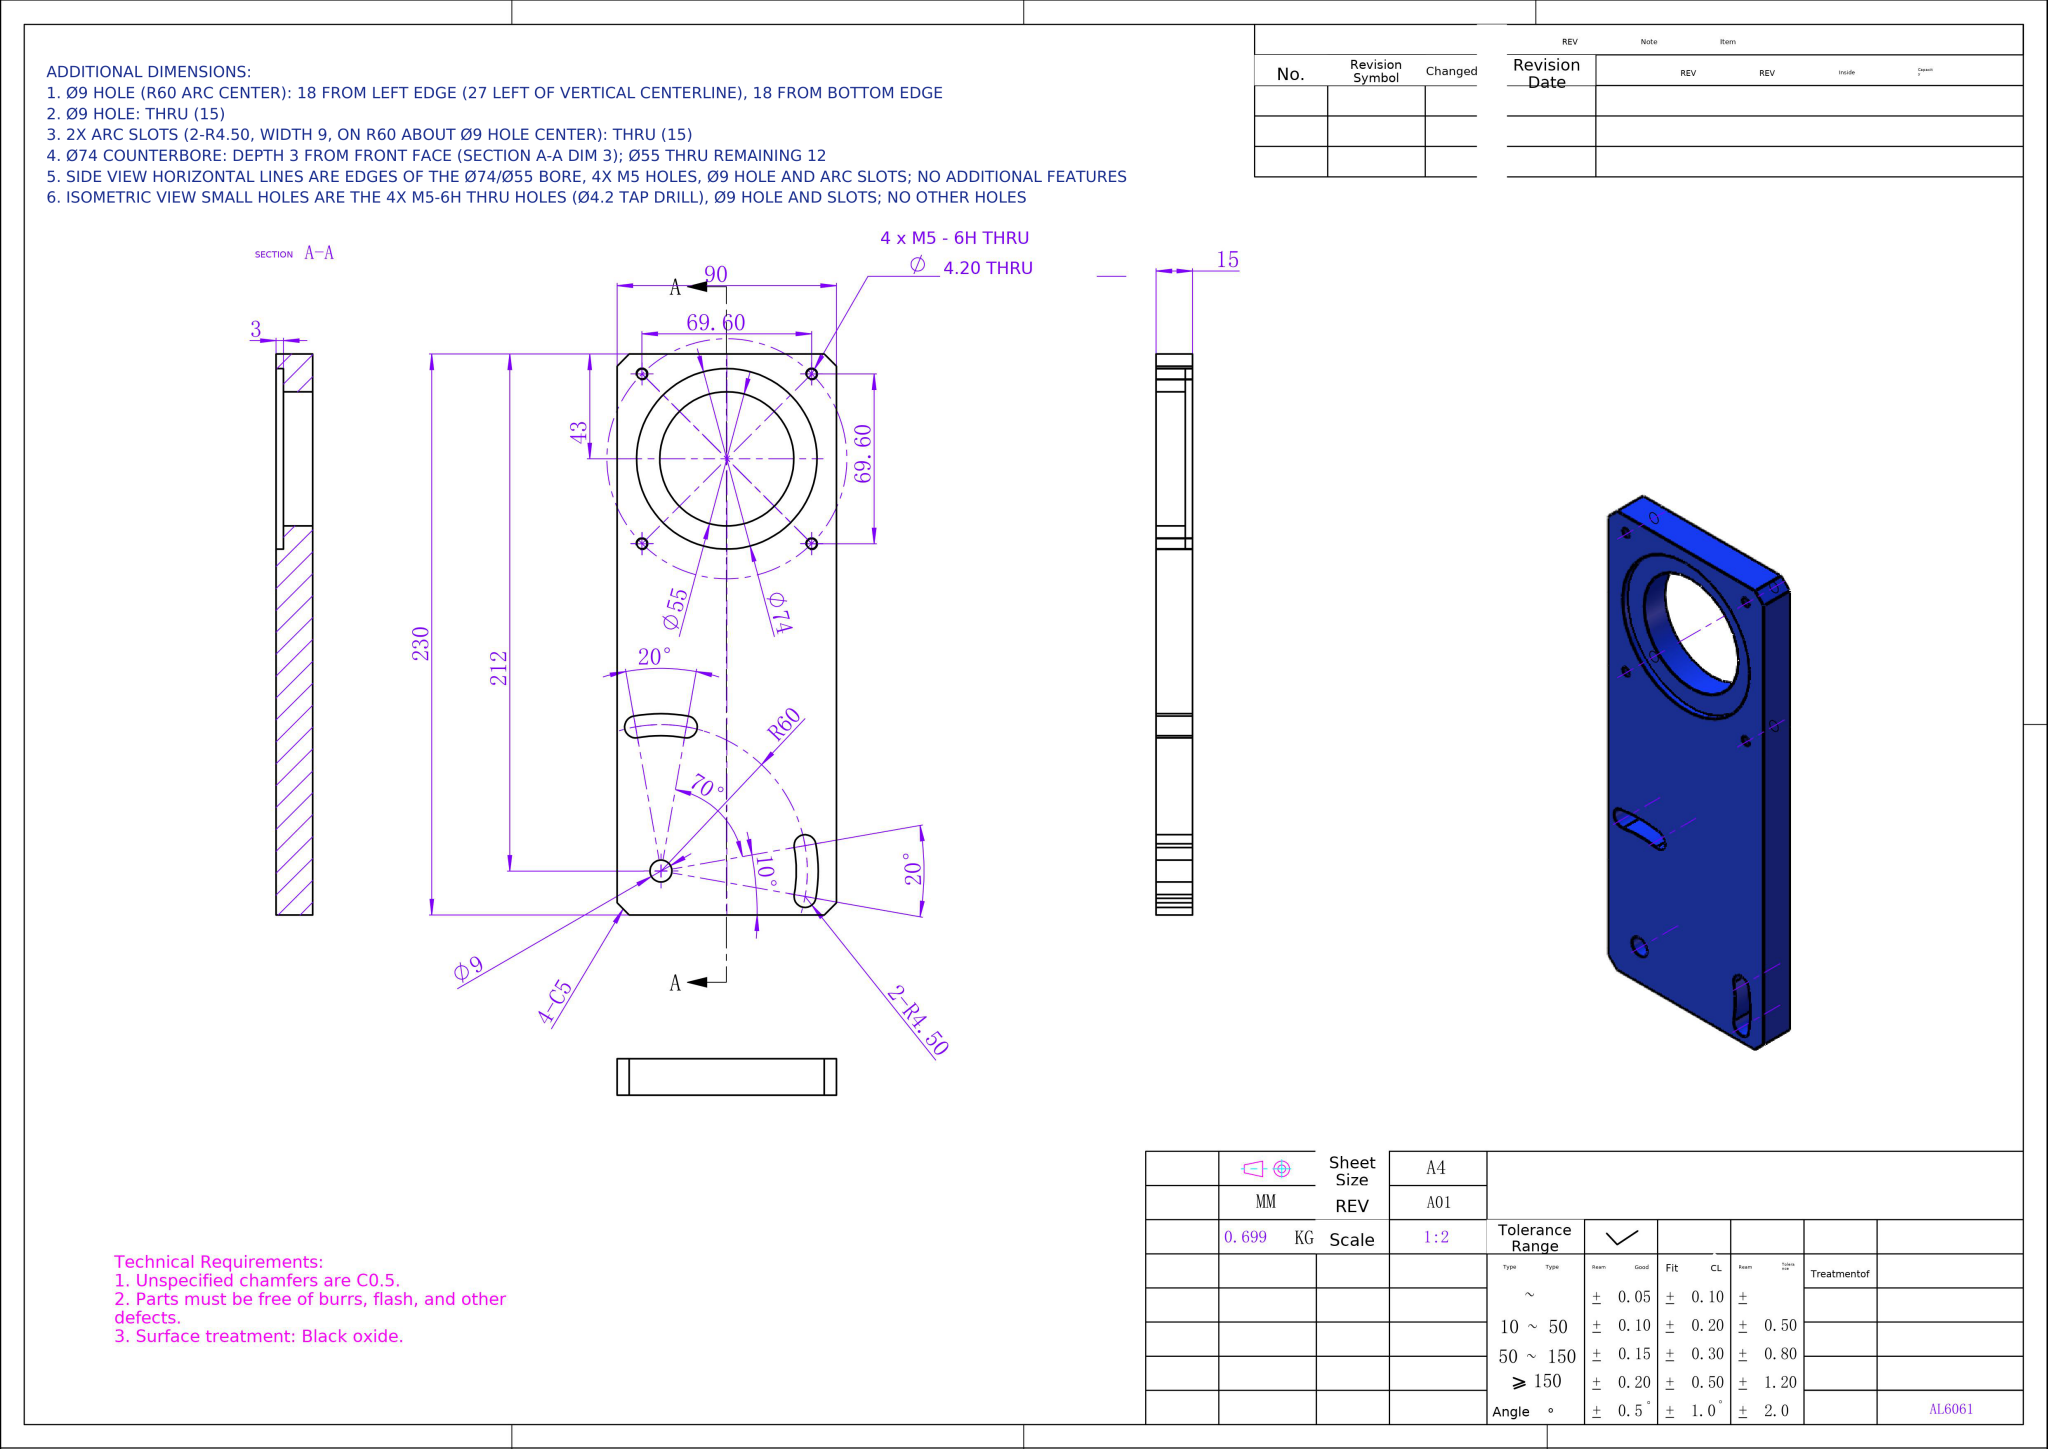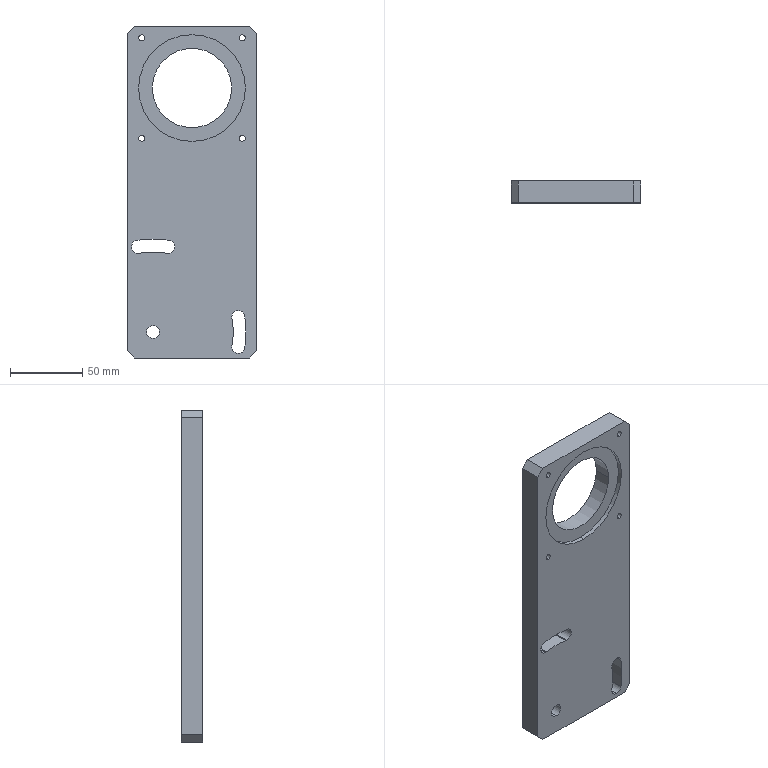Part | NX | mm | 1 solid | 36 faces | box 90 x 15 x 230 mm | volume 258989 mm3 | cylinder 25 | plane 11 | commonest cylinder face diameters 9 x9 4.2 x8 55 x2 74 x2 111 x2 129 x2